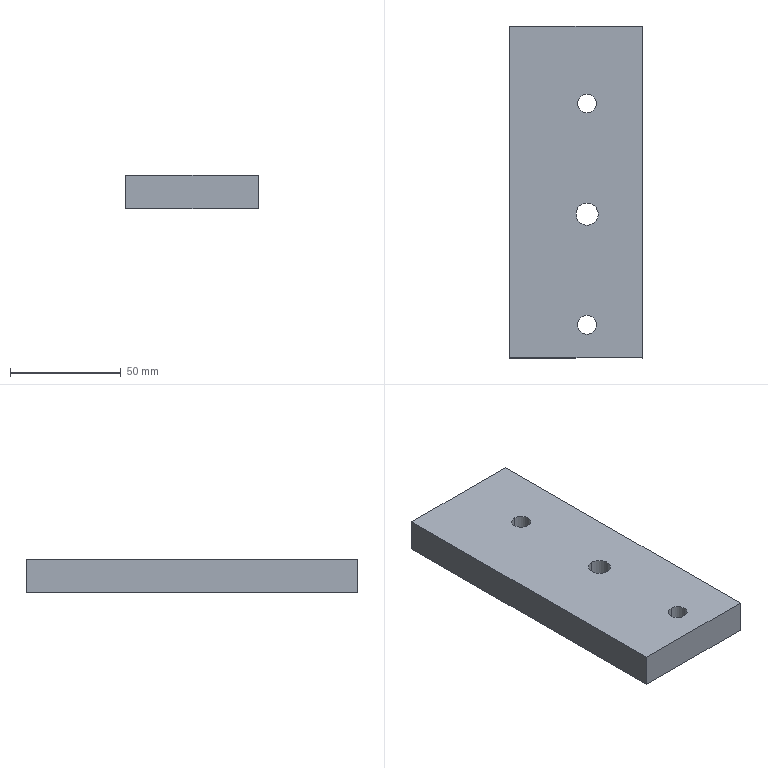Component | SolidWorks | 15mmSteelPlate-331MachineTool-1 | 1 solid | 12 faces | box 60 x 150 x 15 mm | volume 132120 mm3 | cylinder 6 | plane 6 | commonest cylinder face diameters 8.5 x4 10 x2
STEP:
#1=COLOUR_RGB('',0.7922,0.8196,0.9333);
#2=FILL_AREA_STYLE_COLOUR('',#1);
#3=FILL_AREA_STYLE('',(#2));
#4=SURFACE_STYLE_FILL_AREA(#3);
#5=SURFACE_SIDE_STYLE('',(#4));
#6=SURFACE_STYLE_USAGE(.BOTH.,#5);
#7=PRESENTATION_STYLE_ASSIGNMENT((#6));
#8=CARTESIAN_POINT('',(4.635,-2.621,29.724));
#9=VERTEX_POINT('',#8);
#10=CARTESIAN_POINT('',(4.635,-2.227,29.724));
#11=VERTEX_POINT('',#10);
#12=CARTESIAN_POINT('',(4.635,-2.424,29.724));
#13=DIRECTION('',(0.,0.,-1.));
#14=DIRECTION('',(0.,1.,0.));
#15=AXIS2_PLACEMENT_3D('',#12,#13,#14);
#16=CIRCLE('',#15,0.1969);
#17=EDGE_CURVE('',#9,#11,#16,.T.);
#18=ORIENTED_EDGE('',*,*,#17,.F.);
#19=CARTESIAN_POINT('',(4.635,-2.621,29.134));
#20=VERTEX_POINT('',#19);
#21=CARTESIAN_POINT('',(4.635,-2.621,29.134));
#22=DIRECTION('',(0.,0.,-1.));
#23=VECTOR('',#22,39.37);
#24=LINE('',#21,#23);
#25=EDGE_CURVE('',#9,#20,#24,.T.);
#26=ORIENTED_EDGE('',*,*,#25,.T.);
#27=CARTESIAN_POINT('',(4.635,-2.227,29.134));
#28=VERTEX_POINT('',#27);
#29=CARTESIAN_POINT('',(4.635,-2.424,29.134));
#30=DIRECTION('',(0.,0.,-1.));
#31=DIRECTION('',(0.,1.,0.));
#32=AXIS2_PLACEMENT_3D('',#29,#30,#31);
#33=CIRCLE('',#32,0.1969);
#34=EDGE_CURVE('',#20,#28,#33,.T.);
#35=ORIENTED_EDGE('',*,*,#34,.T.);
#36=CARTESIAN_POINT('',(4.635,-2.227,29.134));
#37=DIRECTION('',(0.,0.,-1.));
#38=VECTOR('',#37,39.37);
#39=LINE('',#36,#38);
#40=EDGE_CURVE('',#11,#28,#39,.T.);
#41=ORIENTED_EDGE('',*,*,#40,.F.);
#42=EDGE_LOOP('',(#18,#26,#35,#41));
#43=FACE_OUTER_BOUND('',#42,.T.);
#44=CARTESIAN_POINT('',(4.635,-2.424,29.134));
#45=DIRECTION('',(0.,0.,-1.));
#46=DIRECTION('',(0.,1.,0.));
#47=AXIS2_PLACEMENT_3D('',#44,#45,#46);
#48=CYLINDRICAL_SURFACE('',#47,0.1969);
#49=ADVANCED_FACE('',(#43),#48,.F.);
#50=CARTESIAN_POINT('',(4.635,-0.6225,29.724));
#51=VERTEX_POINT('',#50);
#52=CARTESIAN_POINT('',(4.635,-0.2879,29.724));
#53=VERTEX_POINT('',#52);
#54=CARTESIAN_POINT('',(4.635,-0.4552,29.724));
#55=DIRECTION('',(0.,0.,-1.));
#56=DIRECTION('',(0.,1.,0.));
#57=AXIS2_PLACEMENT_3D('',#54,#55,#56);
#58=CIRCLE('',#57,0.1673);
#59=EDGE_CURVE('',#51,#53,#58,.T.);
#60=ORIENTED_EDGE('',*,*,#59,.F.);
#61=CARTESIAN_POINT('',(4.635,-0.6225,29.134));
#62=VERTEX_POINT('',#61);
#63=CARTESIAN_POINT('',(4.635,-0.6225,29.134));
#64=DIRECTION('',(0.,0.,-1.));
#65=VECTOR('',#64,39.37);
#66=LINE('',#63,#65);
#67=EDGE_CURVE('',#51,#62,#66,.T.);
#68=ORIENTED_EDGE('',*,*,#67,.T.);
#69=CARTESIAN_POINT('',(4.635,-0.2879,29.134));
#70=VERTEX_POINT('',#69);
#71=CARTESIAN_POINT('',(4.635,-0.4552,29.134));
#72=DIRECTION('',(0.,0.,-1.));
#73=DIRECTION('',(0.,1.,0.));
#74=AXIS2_PLACEMENT_3D('',#71,#72,#73);
#75=CIRCLE('',#74,0.1673);
#76=EDGE_CURVE('',#62,#70,#75,.T.);
#77=ORIENTED_EDGE('',*,*,#76,.T.);
#78=CARTESIAN_POINT('',(4.635,-0.2879,29.134));
#79=DIRECTION('',(0.,0.,-1.));
#80=VECTOR('',#79,39.37);
#81=LINE('',#78,#80);
#82=EDGE_CURVE('',#53,#70,#81,.T.);
#83=ORIENTED_EDGE('',*,*,#82,.F.);
#84=EDGE_LOOP('',(#60,#68,#77,#83));
#85=FACE_OUTER_BOUND('',#84,.T.);
#86=CARTESIAN_POINT('',(4.635,-0.4552,29.134));
#87=DIRECTION('',(0.,0.,-1.));
#88=DIRECTION('',(0.,1.,0.));
#89=AXIS2_PLACEMENT_3D('',#86,#87,#88);
#90=CYLINDRICAL_SURFACE('',#89,0.1673);
#91=ADVANCED_FACE('',(#85),#90,.F.);
#92=CARTESIAN_POINT('',(4.635,-4.56,29.724));
#93=VERTEX_POINT('',#92);
#94=CARTESIAN_POINT('',(4.635,-4.225,29.724));
#95=VERTEX_POINT('',#94);
#96=CARTESIAN_POINT('',(4.635,-4.392,29.724));
#97=DIRECTION('',(0.,0.,-1.));
#98=DIRECTION('',(0.,1.,0.));
#99=AXIS2_PLACEMENT_3D('',#96,#97,#98);
#100=CIRCLE('',#99,0.1673);
#101=EDGE_CURVE('',#93,#95,#100,.T.);
#102=ORIENTED_EDGE('',*,*,#101,.F.);
#103=CARTESIAN_POINT('',(4.635,-4.56,29.134));
#104=VERTEX_POINT('',#103);
#105=CARTESIAN_POINT('',(4.635,-4.56,29.134));
#106=DIRECTION('',(0.,0.,-1.));
#107=VECTOR('',#106,39.37);
#108=LINE('',#105,#107);
#109=EDGE_CURVE('',#93,#104,#108,.T.);
#110=ORIENTED_EDGE('',*,*,#109,.T.);
#111=CARTESIAN_POINT('',(4.635,-4.225,29.134));
#112=VERTEX_POINT('',#111);
#113=CARTESIAN_POINT('',(4.635,-4.392,29.134));
#114=DIRECTION('',(0.,0.,-1.));
#115=DIRECTION('',(0.,1.,0.));
#116=AXIS2_PLACEMENT_3D('',#113,#114,#115);
#117=CIRCLE('',#116,0.1673);
#118=EDGE_CURVE('',#104,#112,#117,.T.);
#119=ORIENTED_EDGE('',*,*,#118,.T.);
#120=CARTESIAN_POINT('',(4.635,-4.225,29.134));
#121=DIRECTION('',(0.,0.,-1.));
#122=VECTOR('',#121,39.37);
#123=LINE('',#120,#122);
#124=EDGE_CURVE('',#95,#112,#123,.T.);
#125=ORIENTED_EDGE('',*,*,#124,.F.);
#126=EDGE_LOOP('',(#102,#110,#119,#125));
#127=FACE_OUTER_BOUND('',#126,.T.);
#128=CARTESIAN_POINT('',(4.635,-4.392,29.134));
#129=DIRECTION('',(0.,0.,-1.));
#130=DIRECTION('',(0.,1.,0.));
#131=AXIS2_PLACEMENT_3D('',#128,#129,#130);
#132=CYLINDRICAL_SURFACE('',#131,0.1673);
#133=ADVANCED_FACE('',(#127),#132,.F.);
#134=CARTESIAN_POINT('',(3.257,-4.983,29.134));
#135=VERTEX_POINT('',#134);
#136=CARTESIAN_POINT('',(3.257,0.9228,29.134));
#137=VERTEX_POINT('',#136);
#138=CARTESIAN_POINT('',(3.257,-4.983,29.134));
#139=DIRECTION('',(-0.,1.,0.));
#140=VECTOR('',#139,39.37);
#141=LINE('',#138,#140);
#142=EDGE_CURVE('',#135,#137,#141,.T.);
#143=ORIENTED_EDGE('',*,*,#142,.F.);
#144=CARTESIAN_POINT('',(3.257,-4.983,29.724));
#145=VERTEX_POINT('',#144);
#146=CARTESIAN_POINT('',(3.257,-4.983,29.724));
#147=DIRECTION('',(0.,0.,-1.));
#148=VECTOR('',#147,39.37);
#149=LINE('',#146,#148);
#150=EDGE_CURVE('',#145,#135,#149,.T.);
#151=ORIENTED_EDGE('',*,*,#150,.F.);
#152=CARTESIAN_POINT('',(3.257,0.9228,29.724));
#153=VERTEX_POINT('',#152);
#154=CARTESIAN_POINT('',(3.257,-4.983,29.724));
#155=DIRECTION('',(-0.,1.,0.));
#156=VECTOR('',#155,39.37);
#157=LINE('',#154,#156);
#158=EDGE_CURVE('',#145,#153,#157,.T.);
#159=ORIENTED_EDGE('',*,*,#158,.T.);
#160=CARTESIAN_POINT('',(3.257,0.9228,29.724));
#161=DIRECTION('',(0.,0.,-1.));
#162=VECTOR('',#161,39.37);
#163=LINE('',#160,#162);
#164=EDGE_CURVE('',#153,#137,#163,.T.);
#165=ORIENTED_EDGE('',*,*,#164,.T.);
#166=EDGE_LOOP('',(#143,#151,#159,#165));
#167=FACE_OUTER_BOUND('',#166,.T.);
#168=CARTESIAN_POINT('',(3.257,-4.983,29.724));
#169=DIRECTION('',(-1.,-0.,-0.));
#170=DIRECTION('',(-0.,1.,0.));
#171=AXIS2_PLACEMENT_3D('',#168,#169,#170);
#172=PLANE('',#171);
#173=ADVANCED_FACE('',(#167),#172,.T.);
#174=CARTESIAN_POINT('',(5.619,-4.983,29.134));
#175=VERTEX_POINT('',#174);
#176=CARTESIAN_POINT('',(3.257,-4.983,29.134));
#177=DIRECTION('',(-1.,-0.,-0.));
#178=VECTOR('',#177,39.37);
#179=LINE('',#176,#178);
#180=EDGE_CURVE('',#175,#135,#179,.T.);
#181=ORIENTED_EDGE('',*,*,#180,.F.);
#182=CARTESIAN_POINT('',(5.619,-4.983,29.724));
#183=VERTEX_POINT('',#182);
#184=CARTESIAN_POINT('',(5.619,-4.983,29.724));
#185=DIRECTION('',(0.,0.,-1.));
#186=VECTOR('',#185,39.37);
#187=LINE('',#184,#186);
#188=EDGE_CURVE('',#183,#175,#187,.T.);
#189=ORIENTED_EDGE('',*,*,#188,.F.);
#190=CARTESIAN_POINT('',(3.257,-4.983,29.724));
#191=DIRECTION('',(-1.,-0.,-0.));
#192=VECTOR('',#191,39.37);
#193=LINE('',#190,#192);
#194=EDGE_CURVE('',#183,#145,#193,.T.);
#195=ORIENTED_EDGE('',*,*,#194,.T.);
#196=ORIENTED_EDGE('',*,*,#150,.T.);
#197=EDGE_LOOP('',(#181,#189,#195,#196));
#198=FACE_OUTER_BOUND('',#197,.T.);
#199=CARTESIAN_POINT('',(3.257,-4.983,29.724));
#200=DIRECTION('',(0.,-1.,-0.));
#201=DIRECTION('',(-1.,-0.,-0.));
#202=AXIS2_PLACEMENT_3D('',#199,#200,#201);
#203=PLANE('',#202);
#204=ADVANCED_FACE('',(#198),#203,.T.);
#205=CARTESIAN_POINT('',(5.619,0.9228,29.134));
#206=VERTEX_POINT('',#205);
#207=CARTESIAN_POINT('',(5.619,-4.983,29.134));
#208=DIRECTION('',(0.,-1.,-0.));
#209=VECTOR('',#208,39.37);
#210=LINE('',#207,#209);
#211=EDGE_CURVE('',#206,#175,#210,.T.);
#212=ORIENTED_EDGE('',*,*,#211,.F.);
#213=CARTESIAN_POINT('',(5.619,0.9228,29.724));
#214=VERTEX_POINT('',#213);
#215=CARTESIAN_POINT('',(5.619,0.9228,29.724));
#216=DIRECTION('',(0.,0.,-1.));
#217=VECTOR('',#216,39.37);
#218=LINE('',#215,#217);
#219=EDGE_CURVE('',#214,#206,#218,.T.);
#220=ORIENTED_EDGE('',*,*,#219,.F.);
#221=CARTESIAN_POINT('',(5.619,-4.983,29.724));
#222=DIRECTION('',(0.,-1.,-0.));
#223=VECTOR('',#222,39.37);
#224=LINE('',#221,#223);
#225=EDGE_CURVE('',#214,#183,#224,.T.);
#226=ORIENTED_EDGE('',*,*,#225,.T.);
#227=ORIENTED_EDGE('',*,*,#188,.T.);
#228=EDGE_LOOP('',(#212,#220,#226,#227));
#229=FACE_OUTER_BOUND('',#228,.T.);
#230=CARTESIAN_POINT('',(5.619,-4.983,29.724));
#231=DIRECTION('',(1.,0.,0.));
#232=DIRECTION('',(0.,-1.,-0.));
#233=AXIS2_PLACEMENT_3D('',#230,#231,#232);
#234=PLANE('',#233);
#235=ADVANCED_FACE('',(#229),#234,.T.);
#236=CARTESIAN_POINT('',(3.257,0.9228,29.134));
#237=DIRECTION('',(1.,0.,0.));
#238=VECTOR('',#237,39.37);
#239=LINE('',#236,#238);
#240=EDGE_CURVE('',#137,#206,#239,.T.);
#241=ORIENTED_EDGE('',*,*,#240,.F.);
#242=ORIENTED_EDGE('',*,*,#164,.F.);
#243=CARTESIAN_POINT('',(3.257,0.9228,29.724));
#244=DIRECTION('',(1.,0.,0.));
#245=VECTOR('',#244,39.37);
#246=LINE('',#243,#245);
#247=EDGE_CURVE('',#153,#214,#246,.T.);
#248=ORIENTED_EDGE('',*,*,#247,.T.);
#249=ORIENTED_EDGE('',*,*,#219,.T.);
#250=EDGE_LOOP('',(#241,#242,#248,#249));
#251=FACE_OUTER_BOUND('',#250,.T.);
#252=CARTESIAN_POINT('',(3.257,0.9228,29.724));
#253=DIRECTION('',(-0.,1.,0.));
#254=DIRECTION('',(1.,0.,0.));
#255=AXIS2_PLACEMENT_3D('',#252,#253,#254);
#256=PLANE('',#255);
#257=ADVANCED_FACE('',(#251),#256,.T.);
#258=CARTESIAN_POINT('',(4.635,-2.424,29.724));
#259=DIRECTION('',(0.,0.,-1.));
#260=DIRECTION('',(0.,1.,0.));
#261=AXIS2_PLACEMENT_3D('',#258,#259,#260);
#262=CIRCLE('',#261,0.1969);
#263=EDGE_CURVE('',#11,#9,#262,.T.);
#264=ORIENTED_EDGE('',*,*,#263,.T.);
#265=ORIENTED_EDGE('',*,*,#17,.T.);
#266=EDGE_LOOP('',(#264,#265));
#267=FACE_BOUND('',#266,.T.);
#268=CARTESIAN_POINT('',(4.635,-0.4552,29.724));
#269=DIRECTION('',(0.,0.,-1.));
#270=DIRECTION('',(0.,1.,0.));
#271=AXIS2_PLACEMENT_3D('',#268,#269,#270);
#272=CIRCLE('',#271,0.1673);
#273=EDGE_CURVE('',#53,#51,#272,.T.);
#274=ORIENTED_EDGE('',*,*,#273,.T.);
#275=ORIENTED_EDGE('',*,*,#59,.T.);
#276=EDGE_LOOP('',(#274,#275));
#277=FACE_BOUND('',#276,.T.);
#278=CARTESIAN_POINT('',(4.635,-4.392,29.724));
#279=DIRECTION('',(0.,0.,-1.));
#280=DIRECTION('',(0.,1.,0.));
#281=AXIS2_PLACEMENT_3D('',#278,#279,#280);
#282=CIRCLE('',#281,0.1673);
#283=EDGE_CURVE('',#95,#93,#282,.T.);
#284=ORIENTED_EDGE('',*,*,#283,.T.);
#285=ORIENTED_EDGE('',*,*,#101,.T.);
#286=EDGE_LOOP('',(#284,#285));
#287=FACE_BOUND('',#286,.T.);
#288=ORIENTED_EDGE('',*,*,#158,.F.);
#289=ORIENTED_EDGE('',*,*,#194,.F.);
#290=ORIENTED_EDGE('',*,*,#225,.F.);
#291=ORIENTED_EDGE('',*,*,#247,.F.);
#292=EDGE_LOOP('',(#288,#289,#290,#291));
#293=FACE_OUTER_BOUND('',#292,.T.);
#294=CARTESIAN_POINT('',(5.941,-2.616,29.724));
#295=DIRECTION('',(0.,0.,-1.));
#296=DIRECTION('',(-0.,1.,0.));
#297=AXIS2_PLACEMENT_3D('',#294,#295,#296);
#298=PLANE('',#297);
#299=ADVANCED_FACE('',(#267,#277,#287,#293),#298,.F.);
#300=CARTESIAN_POINT('',(4.635,-2.424,29.134));
#301=DIRECTION('',(0.,0.,-1.));
#302=DIRECTION('',(0.,1.,0.));
#303=AXIS2_PLACEMENT_3D('',#300,#301,#302);
#304=CIRCLE('',#303,0.1969);
#305=EDGE_CURVE('',#28,#20,#304,.T.);
#306=ORIENTED_EDGE('',*,*,#305,.F.);
#307=ORIENTED_EDGE('',*,*,#34,.F.);
#308=EDGE_LOOP('',(#306,#307));
#309=FACE_BOUND('',#308,.T.);
#310=CARTESIAN_POINT('',(4.635,-0.4552,29.134));
#311=DIRECTION('',(0.,0.,-1.));
#312=DIRECTION('',(0.,1.,0.));
#313=AXIS2_PLACEMENT_3D('',#310,#311,#312);
#314=CIRCLE('',#313,0.1673);
#315=EDGE_CURVE('',#70,#62,#314,.T.);
#316=ORIENTED_EDGE('',*,*,#315,.F.);
#317=ORIENTED_EDGE('',*,*,#76,.F.);
#318=EDGE_LOOP('',(#316,#317));
#319=FACE_BOUND('',#318,.T.);
#320=CARTESIAN_POINT('',(4.635,-4.392,29.134));
#321=DIRECTION('',(0.,0.,-1.));
#322=DIRECTION('',(0.,1.,0.));
#323=AXIS2_PLACEMENT_3D('',#320,#321,#322);
#324=CIRCLE('',#323,0.1673);
#325=EDGE_CURVE('',#112,#104,#324,.T.);
#326=ORIENTED_EDGE('',*,*,#325,.F.);
#327=ORIENTED_EDGE('',*,*,#118,.F.);
#328=EDGE_LOOP('',(#326,#327));
#329=FACE_BOUND('',#328,.T.);
#330=ORIENTED_EDGE('',*,*,#142,.T.);
#331=ORIENTED_EDGE('',*,*,#240,.T.);
#332=ORIENTED_EDGE('',*,*,#211,.T.);
#333=ORIENTED_EDGE('',*,*,#180,.T.);
#334=EDGE_LOOP('',(#330,#331,#332,#333));
#335=FACE_OUTER_BOUND('',#334,.T.);
#336=CARTESIAN_POINT('',(5.941,-2.616,29.134));
#337=DIRECTION('',(0.,0.,-1.));
#338=DIRECTION('',(-0.,1.,0.));
#339=AXIS2_PLACEMENT_3D('',#336,#337,#338);
#340=PLANE('',#339);
#341=ADVANCED_FACE('',(#309,#319,#329,#335),#340,.T.);
#342=ORIENTED_EDGE('',*,*,#109,.F.);
#343=ORIENTED_EDGE('',*,*,#283,.F.);
#344=ORIENTED_EDGE('',*,*,#124,.T.);
#345=ORIENTED_EDGE('',*,*,#325,.T.);
#346=EDGE_LOOP('',(#342,#343,#344,#345));
#347=FACE_OUTER_BOUND('',#346,.T.);
#348=CARTESIAN_POINT('',(4.635,-4.392,29.134));
#349=DIRECTION('',(0.,0.,-1.));
#350=DIRECTION('',(0.,1.,0.));
#351=AXIS2_PLACEMENT_3D('',#348,#349,#350);
#352=CYLINDRICAL_SURFACE('',#351,0.1673);
#353=ADVANCED_FACE('',(#347),#352,.F.);
#354=ORIENTED_EDGE('',*,*,#67,.F.);
#355=ORIENTED_EDGE('',*,*,#273,.F.);
#356=ORIENTED_EDGE('',*,*,#82,.T.);
#357=ORIENTED_EDGE('',*,*,#315,.T.);
#358=EDGE_LOOP('',(#354,#355,#356,#357));
#359=FACE_OUTER_BOUND('',#358,.T.);
#360=CARTESIAN_POINT('',(4.635,-0.4552,29.134));
#361=DIRECTION('',(0.,0.,-1.));
#362=DIRECTION('',(0.,1.,0.));
#363=AXIS2_PLACEMENT_3D('',#360,#361,#362);
#364=CYLINDRICAL_SURFACE('',#363,0.1673);
#365=ADVANCED_FACE('',(#359),#364,.F.);
#366=ORIENTED_EDGE('',*,*,#25,.F.);
#367=ORIENTED_EDGE('',*,*,#263,.F.);
#368=ORIENTED_EDGE('',*,*,#40,.T.);
#369=ORIENTED_EDGE('',*,*,#305,.T.);
#370=EDGE_LOOP('',(#366,#367,#368,#369));
#371=FACE_OUTER_BOUND('',#370,.T.);
#372=CARTESIAN_POINT('',(4.635,-2.424,29.134));
#373=DIRECTION('',(0.,0.,-1.));
#374=DIRECTION('',(0.,1.,0.));
#375=AXIS2_PLACEMENT_3D('',#372,#373,#374);
#376=CYLINDRICAL_SURFACE('',#375,0.1969);
#377=ADVANCED_FACE('',(#371),#376,.F.);
#378=CLOSED_SHELL('',(#49,#91,#133,#173,#204,#235,#257,#299,#341,#353,#365,#377));
#379=MANIFOLD_SOLID_BREP('',#378);
#380=STYLED_ITEM('',(#7),#379);
#381=(LENGTH_UNIT()NAMED_UNIT(*)SI_UNIT($,.METRE.));
#382=LENGTH_MEASURE_WITH_UNIT(LENGTH_MEASURE(0.0254),#381);
#383=DIMENSIONAL_EXPONENTS(1.,0.,0.,0.,0.,0.,0.);
#384=(CONVERSION_BASED_UNIT('',#382)LENGTH_UNIT()NAMED_UNIT(#383));
#385=UNCERTAINTY_MEASURE_WITH_UNIT(LENGTH_MEASURE(0.00001),#384,'','');
#386=(NAMED_UNIT(*)PLANE_ANGLE_UNIT()SI_UNIT($,.RADIAN.));
#387=(NAMED_UNIT(*)SI_UNIT($,.STERADIAN.)SOLID_ANGLE_UNIT());
#388=(GEOMETRIC_REPRESENTATION_CONTEXT(3)GLOBAL_UNCERTAINTY_ASSIGNED_CONTEXT((#385))GLOBAL_UNIT_ASSIGNED_CONTEXT((#384,#386,#387))REPRESENTATION_CONTEXT('',''));
#389=MECHANICAL_DESIGN_GEOMETRIC_PRESENTATION_REPRESENTATION('',(#380),#388);
#390=PRESENTATION_LAYER_ASSIGNMENT('','',(#380));
#391=CARTESIAN_POINT('',(0.,0.,0.));
#392=DIRECTION('',(0.,0.,1.));
#393=DIRECTION('',(1.,0.,0.));
#394=AXIS2_PLACEMENT_3D('',#391,#392,#393);
#395=(LENGTH_UNIT()NAMED_UNIT(*)SI_UNIT($,.METRE.));
#396=LENGTH_MEASURE_WITH_UNIT(LENGTH_MEASURE(0.0254),#395);
#397=DIMENSIONAL_EXPONENTS(1.,0.,0.,0.,0.,0.,0.);
#398=(CONVERSION_BASED_UNIT('',#396)LENGTH_UNIT()NAMED_UNIT(#397));
#399=UNCERTAINTY_MEASURE_WITH_UNIT(LENGTH_MEASURE(0.00001),#398,'','');
#400=(NAMED_UNIT(*)PLANE_ANGLE_UNIT()SI_UNIT($,.RADIAN.));
#401=(NAMED_UNIT(*)SI_UNIT($,.STERADIAN.)SOLID_ANGLE_UNIT());
#402=(GEOMETRIC_REPRESENTATION_CONTEXT(3)GLOBAL_UNCERTAINTY_ASSIGNED_CONTEXT((#399))GLOBAL_UNIT_ASSIGNED_CONTEXT((#398,#400,#401))REPRESENTATION_CONTEXT('',''));
#403=ADVANCED_BREP_SHAPE_REPRESENTATION('',(#379,#394),#402);